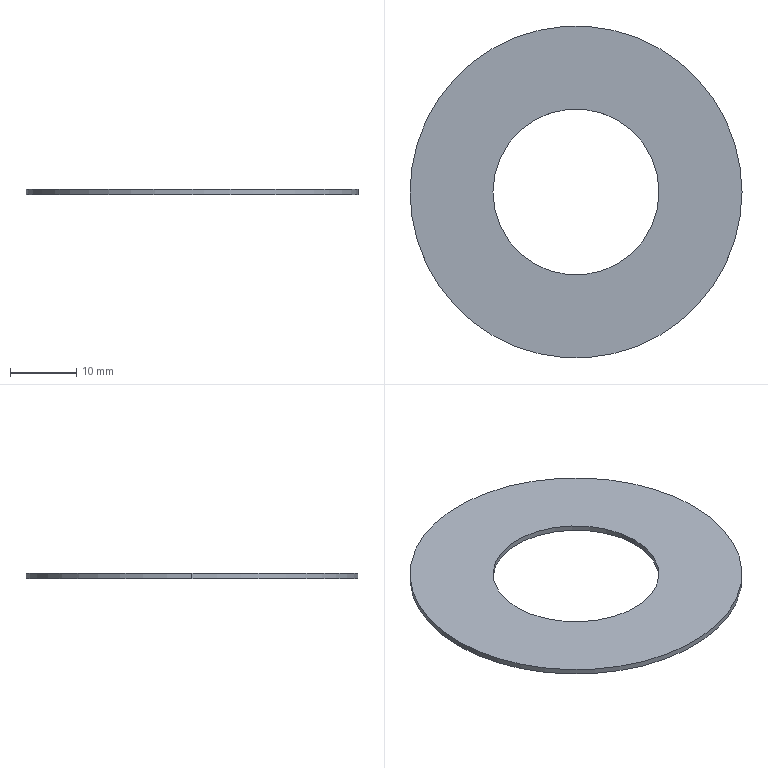Component | SolidWorks | 0.8Gasket0-10 | 1 solid | 6 faces | box 50 x 50 x 0.8 mm | volume 1178 mm3 | cylinder 4 | plane 2 | commonest cylinder face diameters 25 x2 50 x2
build123d program:
from build123d import *

# Parameters (mm, degrees)
SKETCH1_R           = 25
SKETCH1_R_2         = 12.5
BOSS_EXTRUDE1_DEPTH = 0.8


with BuildPart() as part:
    # Sketch1 → Boss-Extrude1 (new body)
    with BuildSketch(Plane.XY):
        Circle(SKETCH1_R)
        Circle(SKETCH1_R_2, mode=Mode.SUBTRACT)
    extrude(amount=BOSS_EXTRUDE1_DEPTH)


solid = part.part

# Placed as in the assembly
solid = solid.moved(Location((-15.093, -37.782, 233.455), (0, 0, 0)))